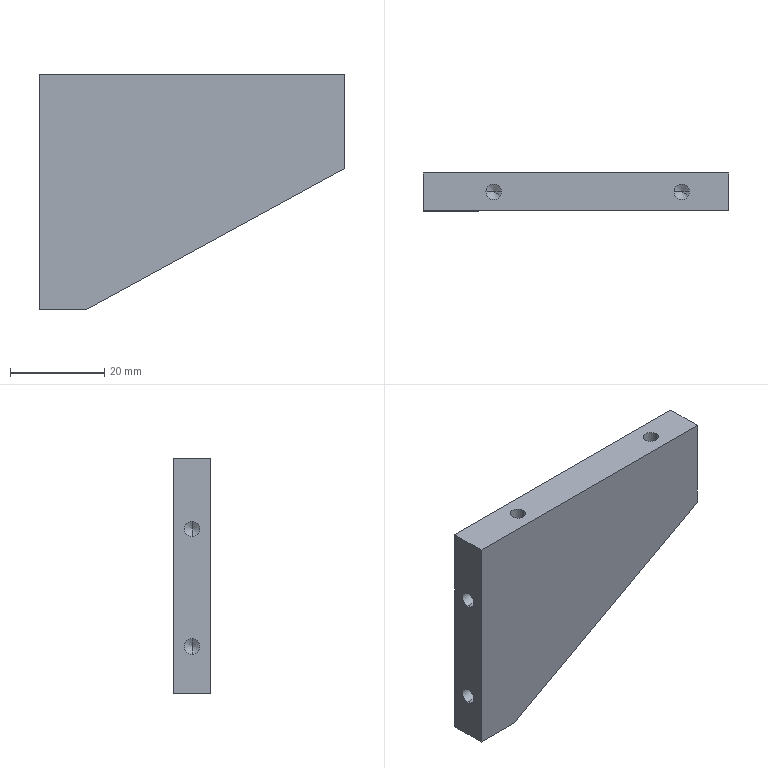CAM job | Mastercam | mm | 6 operations | part box 65 x 8 x 50
1. Drill/Counterbore | 2 - 6定位倒角
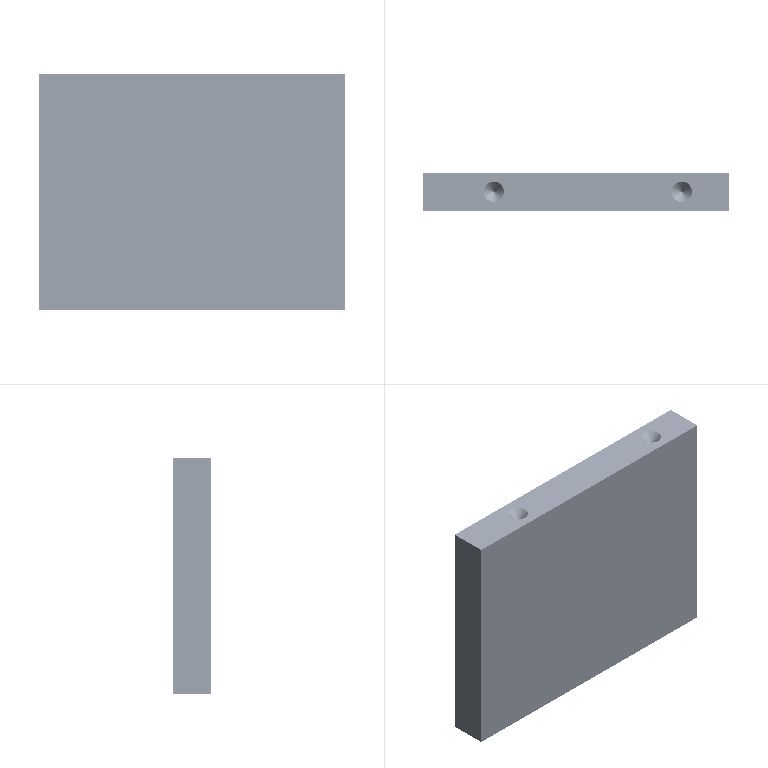2. Peck Drill | 12 - 3.3 钻头
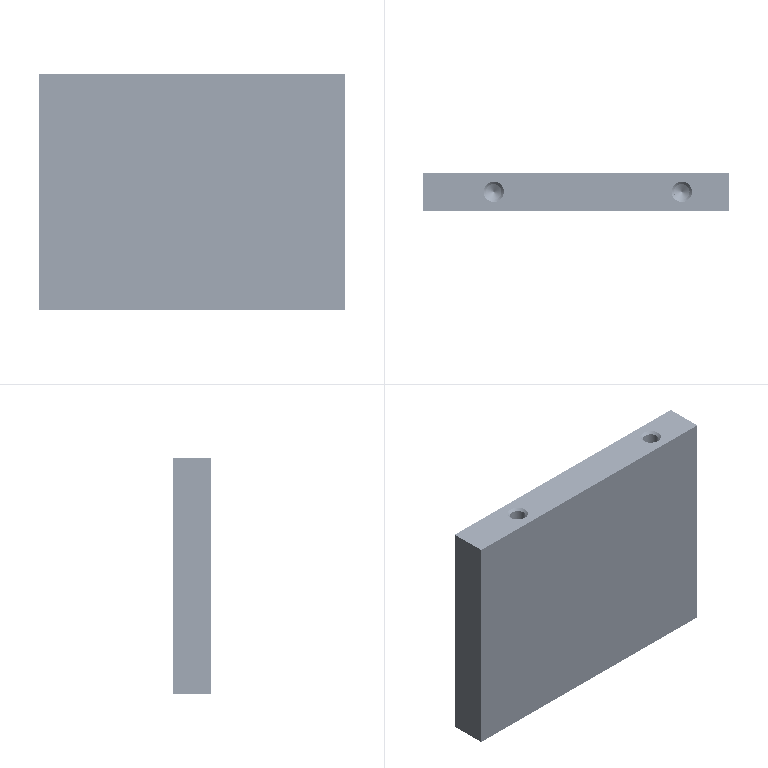3. Thread Mill | 20 - M4/0.7-3.15 螺纹铣刀
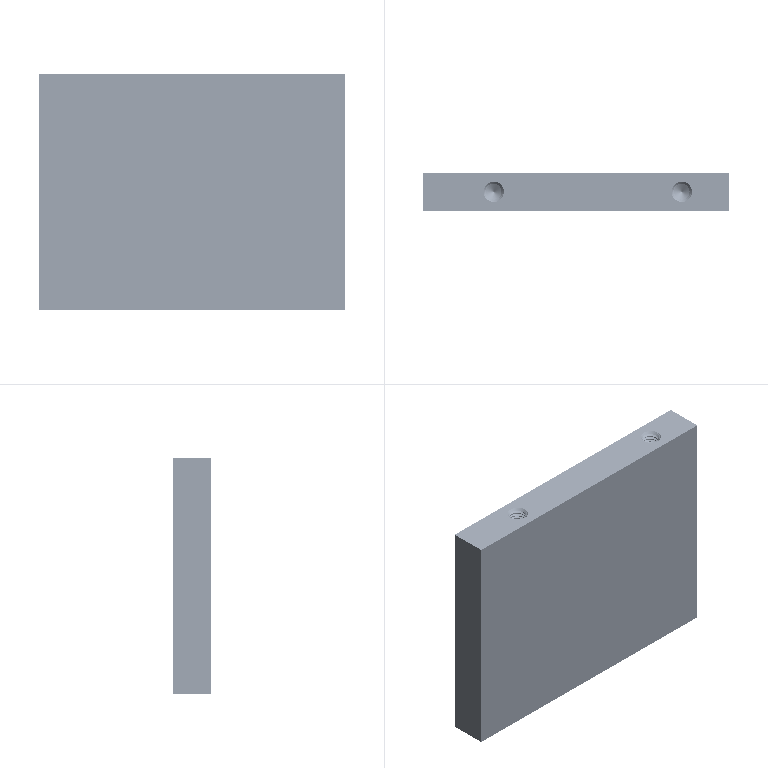4. Drill/Counterbore | 2 - 6定位倒角
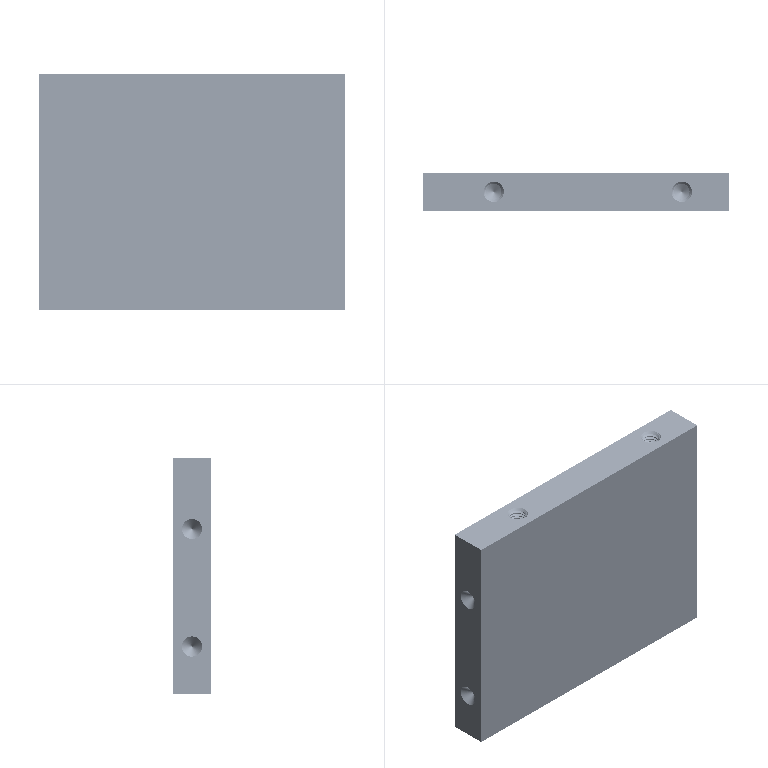5. Peck Drill | 12 - 3.3 钻头
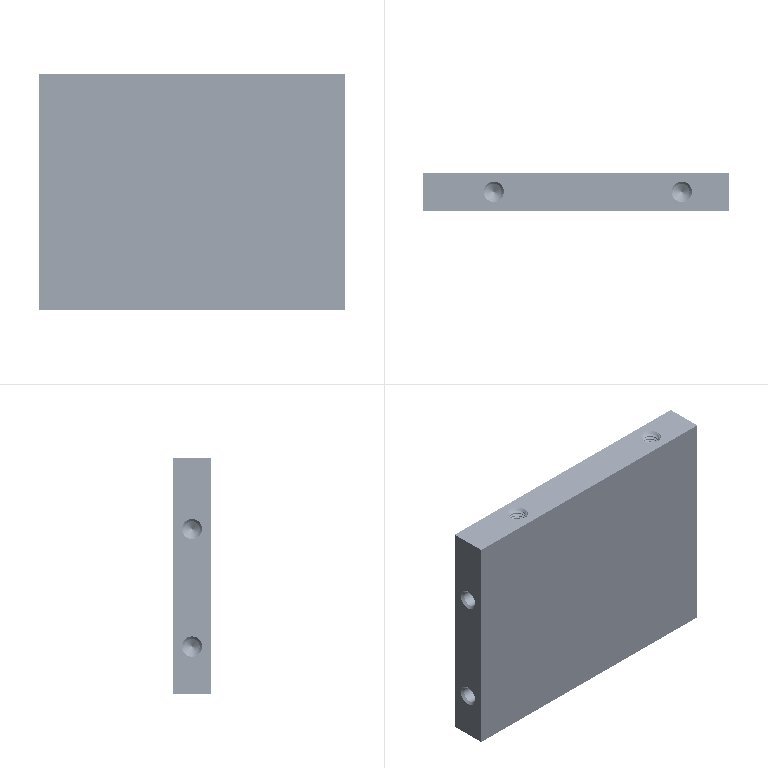6. Thread Mill | 20 - M4/0.7-3.15 螺纹铣刀